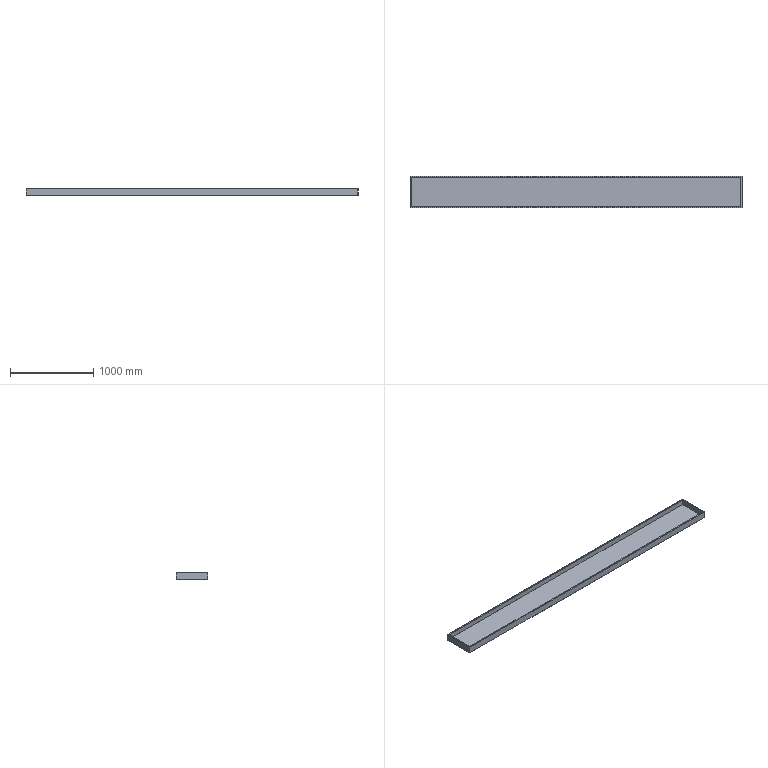Component | NX | DB9 | 1 solid | 16 faces | volume 3478377 mm3 | plane 16